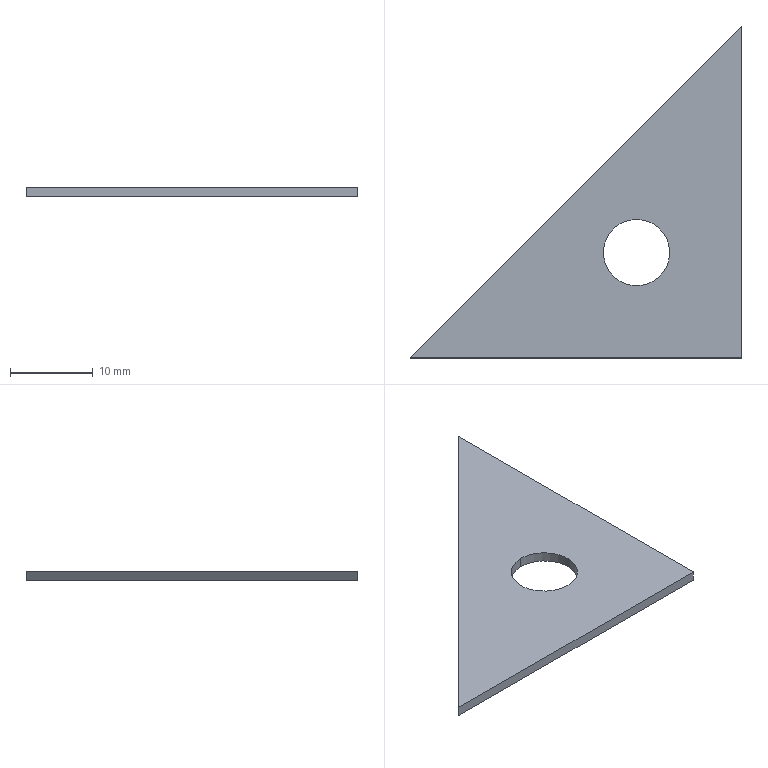Component | SolidWorks | WeldmentDrawing-1_MountingAngle-1 | 1 solid | 7 faces | box 40 x 40 x 1.2 mm | volume 900 mm3 | plane 5 | cylinder 2 | commonest cylinder face diameters 8 x2
STEP:
#1=CARTESIAN_POINT('',(4.789,-3.719,9.055));
#2=VERTEX_POINT('',#1);
#3=CARTESIAN_POINT('',(4.789,-3.404,9.055));
#4=VERTEX_POINT('',#3);
#5=CARTESIAN_POINT('',(4.789,-3.561,9.055));
#6=DIRECTION('',(0.,-0.,1.));
#7=DIRECTION('',(0.,1.,0.));
#8=AXIS2_PLACEMENT_3D('',#5,#6,#7);
#9=CIRCLE('',#8,0.1575);
#10=EDGE_CURVE('',#2,#4,#9,.T.);
#11=ORIENTED_EDGE('',*,*,#10,.F.);
#12=CARTESIAN_POINT('',(4.789,-3.719,9.102));
#13=VERTEX_POINT('',#12);
#14=CARTESIAN_POINT('',(4.789,-3.719,9.055));
#15=DIRECTION('',(0.,-0.,1.));
#16=VECTOR('',#15,39.37);
#17=LINE('',#14,#16);
#18=EDGE_CURVE('',#2,#13,#17,.T.);
#19=ORIENTED_EDGE('',*,*,#18,.T.);
#20=CARTESIAN_POINT('',(4.789,-3.404,9.102));
#21=VERTEX_POINT('',#20);
#22=CARTESIAN_POINT('',(4.789,-3.561,9.102));
#23=DIRECTION('',(0.,-0.,1.));
#24=DIRECTION('',(0.,1.,0.));
#25=AXIS2_PLACEMENT_3D('',#22,#23,#24);
#26=CIRCLE('',#25,0.1575);
#27=EDGE_CURVE('',#13,#21,#26,.T.);
#28=ORIENTED_EDGE('',*,*,#27,.T.);
#29=CARTESIAN_POINT('',(4.789,-3.404,9.055));
#30=DIRECTION('',(0.,-0.,1.));
#31=VECTOR('',#30,39.37);
#32=LINE('',#29,#31);
#33=EDGE_CURVE('',#4,#21,#32,.T.);
#34=ORIENTED_EDGE('',*,*,#33,.F.);
#35=EDGE_LOOP('',(#11,#19,#28,#34));
#36=FACE_OUTER_BOUND('',#35,.T.);
#37=CARTESIAN_POINT('',(4.789,-3.561,9.055));
#38=DIRECTION('',(0.,-0.,1.));
#39=DIRECTION('',(0.,1.,0.));
#40=AXIS2_PLACEMENT_3D('',#37,#38,#39);
#41=CYLINDRICAL_SURFACE('',#40,0.1575);
#42=ADVANCED_FACE('',(#36),#41,.F.);
#43=CARTESIAN_POINT('',(5.289,-2.486,9.102));
#44=VERTEX_POINT('',#43);
#45=CARTESIAN_POINT('',(3.714,-4.061,9.102));
#46=VERTEX_POINT('',#45);
#47=CARTESIAN_POINT('',(5.289,-2.486,9.102));
#48=DIRECTION('',(-0.7071,-0.7071,-0.));
#49=VECTOR('',#48,39.37);
#50=LINE('',#47,#49);
#51=EDGE_CURVE('',#44,#46,#50,.T.);
#52=ORIENTED_EDGE('',*,*,#51,.F.);
#53=CARTESIAN_POINT('',(5.289,-2.486,9.055));
#54=VERTEX_POINT('',#53);
#55=CARTESIAN_POINT('',(5.289,-2.486,9.055));
#56=DIRECTION('',(0.,-0.,1.));
#57=VECTOR('',#56,39.37);
#58=LINE('',#55,#57);
#59=EDGE_CURVE('',#54,#44,#58,.T.);
#60=ORIENTED_EDGE('',*,*,#59,.F.);
#61=CARTESIAN_POINT('',(3.714,-4.061,9.055));
#62=VERTEX_POINT('',#61);
#63=CARTESIAN_POINT('',(5.289,-2.486,9.055));
#64=DIRECTION('',(-0.7071,-0.7071,-0.));
#65=VECTOR('',#64,39.37);
#66=LINE('',#63,#65);
#67=EDGE_CURVE('',#54,#62,#66,.T.);
#68=ORIENTED_EDGE('',*,*,#67,.T.);
#69=CARTESIAN_POINT('',(3.714,-4.061,9.055));
#70=DIRECTION('',(0.,-0.,1.));
#71=VECTOR('',#70,39.37);
#72=LINE('',#69,#71);
#73=EDGE_CURVE('',#62,#46,#72,.T.);
#74=ORIENTED_EDGE('',*,*,#73,.T.);
#75=EDGE_LOOP('',(#52,#60,#68,#74));
#76=FACE_OUTER_BOUND('',#75,.T.);
#77=CARTESIAN_POINT('',(5.289,-2.486,9.055));
#78=DIRECTION('',(-0.7071,0.7071,0.));
#79=DIRECTION('',(-0.7071,-0.7071,-0.));
#80=AXIS2_PLACEMENT_3D('',#77,#78,#79);
#81=PLANE('',#80);
#82=ADVANCED_FACE('',(#76),#81,.T.);
#83=CARTESIAN_POINT('',(5.289,-4.061,9.102));
#84=VERTEX_POINT('',#83);
#85=CARTESIAN_POINT('',(5.289,-4.061,9.102));
#86=DIRECTION('',(0.,1.,0.));
#87=VECTOR('',#86,39.37);
#88=LINE('',#85,#87);
#89=EDGE_CURVE('',#84,#44,#88,.T.);
#90=ORIENTED_EDGE('',*,*,#89,.F.);
#91=CARTESIAN_POINT('',(5.289,-4.061,9.055));
#92=VERTEX_POINT('',#91);
#93=CARTESIAN_POINT('',(5.289,-4.061,9.055));
#94=DIRECTION('',(0.,-0.,1.));
#95=VECTOR('',#94,39.37);
#96=LINE('',#93,#95);
#97=EDGE_CURVE('',#92,#84,#96,.T.);
#98=ORIENTED_EDGE('',*,*,#97,.F.);
#99=CARTESIAN_POINT('',(5.289,-4.061,9.055));
#100=DIRECTION('',(0.,1.,0.));
#101=VECTOR('',#100,39.37);
#102=LINE('',#99,#101);
#103=EDGE_CURVE('',#92,#54,#102,.T.);
#104=ORIENTED_EDGE('',*,*,#103,.T.);
#105=ORIENTED_EDGE('',*,*,#59,.T.);
#106=EDGE_LOOP('',(#90,#98,#104,#105));
#107=FACE_OUTER_BOUND('',#106,.T.);
#108=CARTESIAN_POINT('',(5.289,-4.061,9.055));
#109=DIRECTION('',(1.,0.,-0.));
#110=DIRECTION('',(-0.,0.,-1.));
#111=AXIS2_PLACEMENT_3D('',#108,#109,#110);
#112=PLANE('',#111);
#113=ADVANCED_FACE('',(#107),#112,.T.);
#114=CARTESIAN_POINT('',(3.714,-4.061,9.102));
#115=DIRECTION('',(1.,0.,-0.));
#116=VECTOR('',#115,39.37);
#117=LINE('',#114,#116);
#118=EDGE_CURVE('',#46,#84,#117,.T.);
#119=ORIENTED_EDGE('',*,*,#118,.F.);
#120=ORIENTED_EDGE('',*,*,#73,.F.);
#121=CARTESIAN_POINT('',(3.714,-4.061,9.055));
#122=DIRECTION('',(1.,0.,-0.));
#123=VECTOR('',#122,39.37);
#124=LINE('',#121,#123);
#125=EDGE_CURVE('',#62,#92,#124,.T.);
#126=ORIENTED_EDGE('',*,*,#125,.T.);
#127=ORIENTED_EDGE('',*,*,#97,.T.);
#128=EDGE_LOOP('',(#119,#120,#126,#127));
#129=FACE_OUTER_BOUND('',#128,.T.);
#130=CARTESIAN_POINT('',(3.714,-4.061,9.055));
#131=DIRECTION('',(0.,-1.,-0.));
#132=DIRECTION('',(1.,0.,-0.));
#133=AXIS2_PLACEMENT_3D('',#130,#131,#132);
#134=PLANE('',#133);
#135=ADVANCED_FACE('',(#129),#134,.T.);
#136=CARTESIAN_POINT('',(4.789,-3.561,9.055));
#137=DIRECTION('',(0.,-0.,1.));
#138=DIRECTION('',(0.,1.,0.));
#139=AXIS2_PLACEMENT_3D('',#136,#137,#138);
#140=CIRCLE('',#139,0.1575);
#141=EDGE_CURVE('',#4,#2,#140,.T.);
#142=ORIENTED_EDGE('',*,*,#141,.T.);
#143=ORIENTED_EDGE('',*,*,#10,.T.);
#144=EDGE_LOOP('',(#142,#143));
#145=FACE_BOUND('',#144,.T.);
#146=ORIENTED_EDGE('',*,*,#67,.F.);
#147=ORIENTED_EDGE('',*,*,#103,.F.);
#148=ORIENTED_EDGE('',*,*,#125,.F.);
#149=EDGE_LOOP('',(#146,#147,#148));
#150=FACE_OUTER_BOUND('',#149,.T.);
#151=CARTESIAN_POINT('',(5.932,-2.493,9.055));
#152=DIRECTION('',(0.,-0.,1.));
#153=DIRECTION('',(0.,1.,0.));
#154=AXIS2_PLACEMENT_3D('',#151,#152,#153);
#155=PLANE('',#154);
#156=ADVANCED_FACE('',(#145,#150),#155,.F.);
#157=CARTESIAN_POINT('',(4.789,-3.561,9.102));
#158=DIRECTION('',(0.,-0.,1.));
#159=DIRECTION('',(0.,1.,0.));
#160=AXIS2_PLACEMENT_3D('',#157,#158,#159);
#161=CIRCLE('',#160,0.1575);
#162=EDGE_CURVE('',#21,#13,#161,.T.);
#163=ORIENTED_EDGE('',*,*,#162,.F.);
#164=ORIENTED_EDGE('',*,*,#27,.F.);
#165=EDGE_LOOP('',(#163,#164));
#166=FACE_BOUND('',#165,.T.);
#167=ORIENTED_EDGE('',*,*,#51,.T.);
#168=ORIENTED_EDGE('',*,*,#118,.T.);
#169=ORIENTED_EDGE('',*,*,#89,.T.);
#170=EDGE_LOOP('',(#167,#168,#169));
#171=FACE_OUTER_BOUND('',#170,.T.);
#172=CARTESIAN_POINT('',(5.932,-2.493,9.102));
#173=DIRECTION('',(0.,-0.,1.));
#174=DIRECTION('',(0.,1.,0.));
#175=AXIS2_PLACEMENT_3D('',#172,#173,#174);
#176=PLANE('',#175);
#177=ADVANCED_FACE('',(#166,#171),#176,.T.);
#178=ORIENTED_EDGE('',*,*,#18,.F.);
#179=ORIENTED_EDGE('',*,*,#141,.F.);
#180=ORIENTED_EDGE('',*,*,#33,.T.);
#181=ORIENTED_EDGE('',*,*,#162,.T.);
#182=EDGE_LOOP('',(#178,#179,#180,#181));
#183=FACE_OUTER_BOUND('',#182,.T.);
#184=CARTESIAN_POINT('',(4.789,-3.561,9.055));
#185=DIRECTION('',(0.,-0.,1.));
#186=DIRECTION('',(0.,1.,0.));
#187=AXIS2_PLACEMENT_3D('',#184,#185,#186);
#188=CYLINDRICAL_SURFACE('',#187,0.1575);
#189=ADVANCED_FACE('',(#183),#188,.F.);
#190=CLOSED_SHELL('',(#42,#82,#113,#135,#156,#177,#189));
#191=MANIFOLD_SOLID_BREP('',#190);
#192=CARTESIAN_POINT('',(0.,0.,0.));
#193=DIRECTION('',(0.,0.,1.));
#194=DIRECTION('',(1.,0.,0.));
#195=AXIS2_PLACEMENT_3D('',#192,#193,#194);
#196=(LENGTH_UNIT()NAMED_UNIT(*)SI_UNIT($,.METRE.));
#197=LENGTH_MEASURE_WITH_UNIT(LENGTH_MEASURE(0.0254),#196);
#198=DIMENSIONAL_EXPONENTS(1.,0.,0.,0.,0.,0.,0.);
#199=(CONVERSION_BASED_UNIT('',#197)LENGTH_UNIT()NAMED_UNIT(#198));
#200=UNCERTAINTY_MEASURE_WITH_UNIT(LENGTH_MEASURE(0.00001),#199,'','');
#201=(NAMED_UNIT(*)PLANE_ANGLE_UNIT()SI_UNIT($,.RADIAN.));
#202=(NAMED_UNIT(*)SI_UNIT($,.STERADIAN.)SOLID_ANGLE_UNIT());
#203=(GEOMETRIC_REPRESENTATION_CONTEXT(3)GLOBAL_UNCERTAINTY_ASSIGNED_CONTEXT((#200))GLOBAL_UNIT_ASSIGNED_CONTEXT((#199,#201,#202))REPRESENTATION_CONTEXT('',''));
#204=ADVANCED_BREP_SHAPE_REPRESENTATION('',(#191,#195),#203);
#205=COLOUR_RGB('',0.7922,0.8196,0.9333);
#206=FILL_AREA_STYLE_COLOUR('',#205);
#207=FILL_AREA_STYLE('',(#206));
#208=SURFACE_STYLE_FILL_AREA(#207);
#209=SURFACE_SIDE_STYLE('',(#208));
#210=SURFACE_STYLE_USAGE(.BOTH.,#209);
#211=PRESENTATION_STYLE_ASSIGNMENT((#210));
#212=STYLED_ITEM('',(#211),#191);
#213=PRESENTATION_LAYER_ASSIGNMENT('','',(#212));
#214=(LENGTH_UNIT()NAMED_UNIT(*)SI_UNIT($,.METRE.));
#215=LENGTH_MEASURE_WITH_UNIT(LENGTH_MEASURE(0.0254),#214);
#216=DIMENSIONAL_EXPONENTS(1.,0.,0.,0.,0.,0.,0.);
#217=(CONVERSION_BASED_UNIT('',#215)LENGTH_UNIT()NAMED_UNIT(#216));
#218=UNCERTAINTY_MEASURE_WITH_UNIT(LENGTH_MEASURE(0.00001),#217,'','');
#219=(NAMED_UNIT(*)PLANE_ANGLE_UNIT()SI_UNIT($,.RADIAN.));
#220=(NAMED_UNIT(*)SI_UNIT($,.STERADIAN.)SOLID_ANGLE_UNIT());
#221=(GEOMETRIC_REPRESENTATION_CONTEXT(3)GLOBAL_UNCERTAINTY_ASSIGNED_CONTEXT((#218))GLOBAL_UNIT_ASSIGNED_CONTEXT((#217,#219,#220))REPRESENTATION_CONTEXT('',''));
#222=MECHANICAL_DESIGN_GEOMETRIC_PRESENTATION_REPRESENTATION('',(#212),#221);